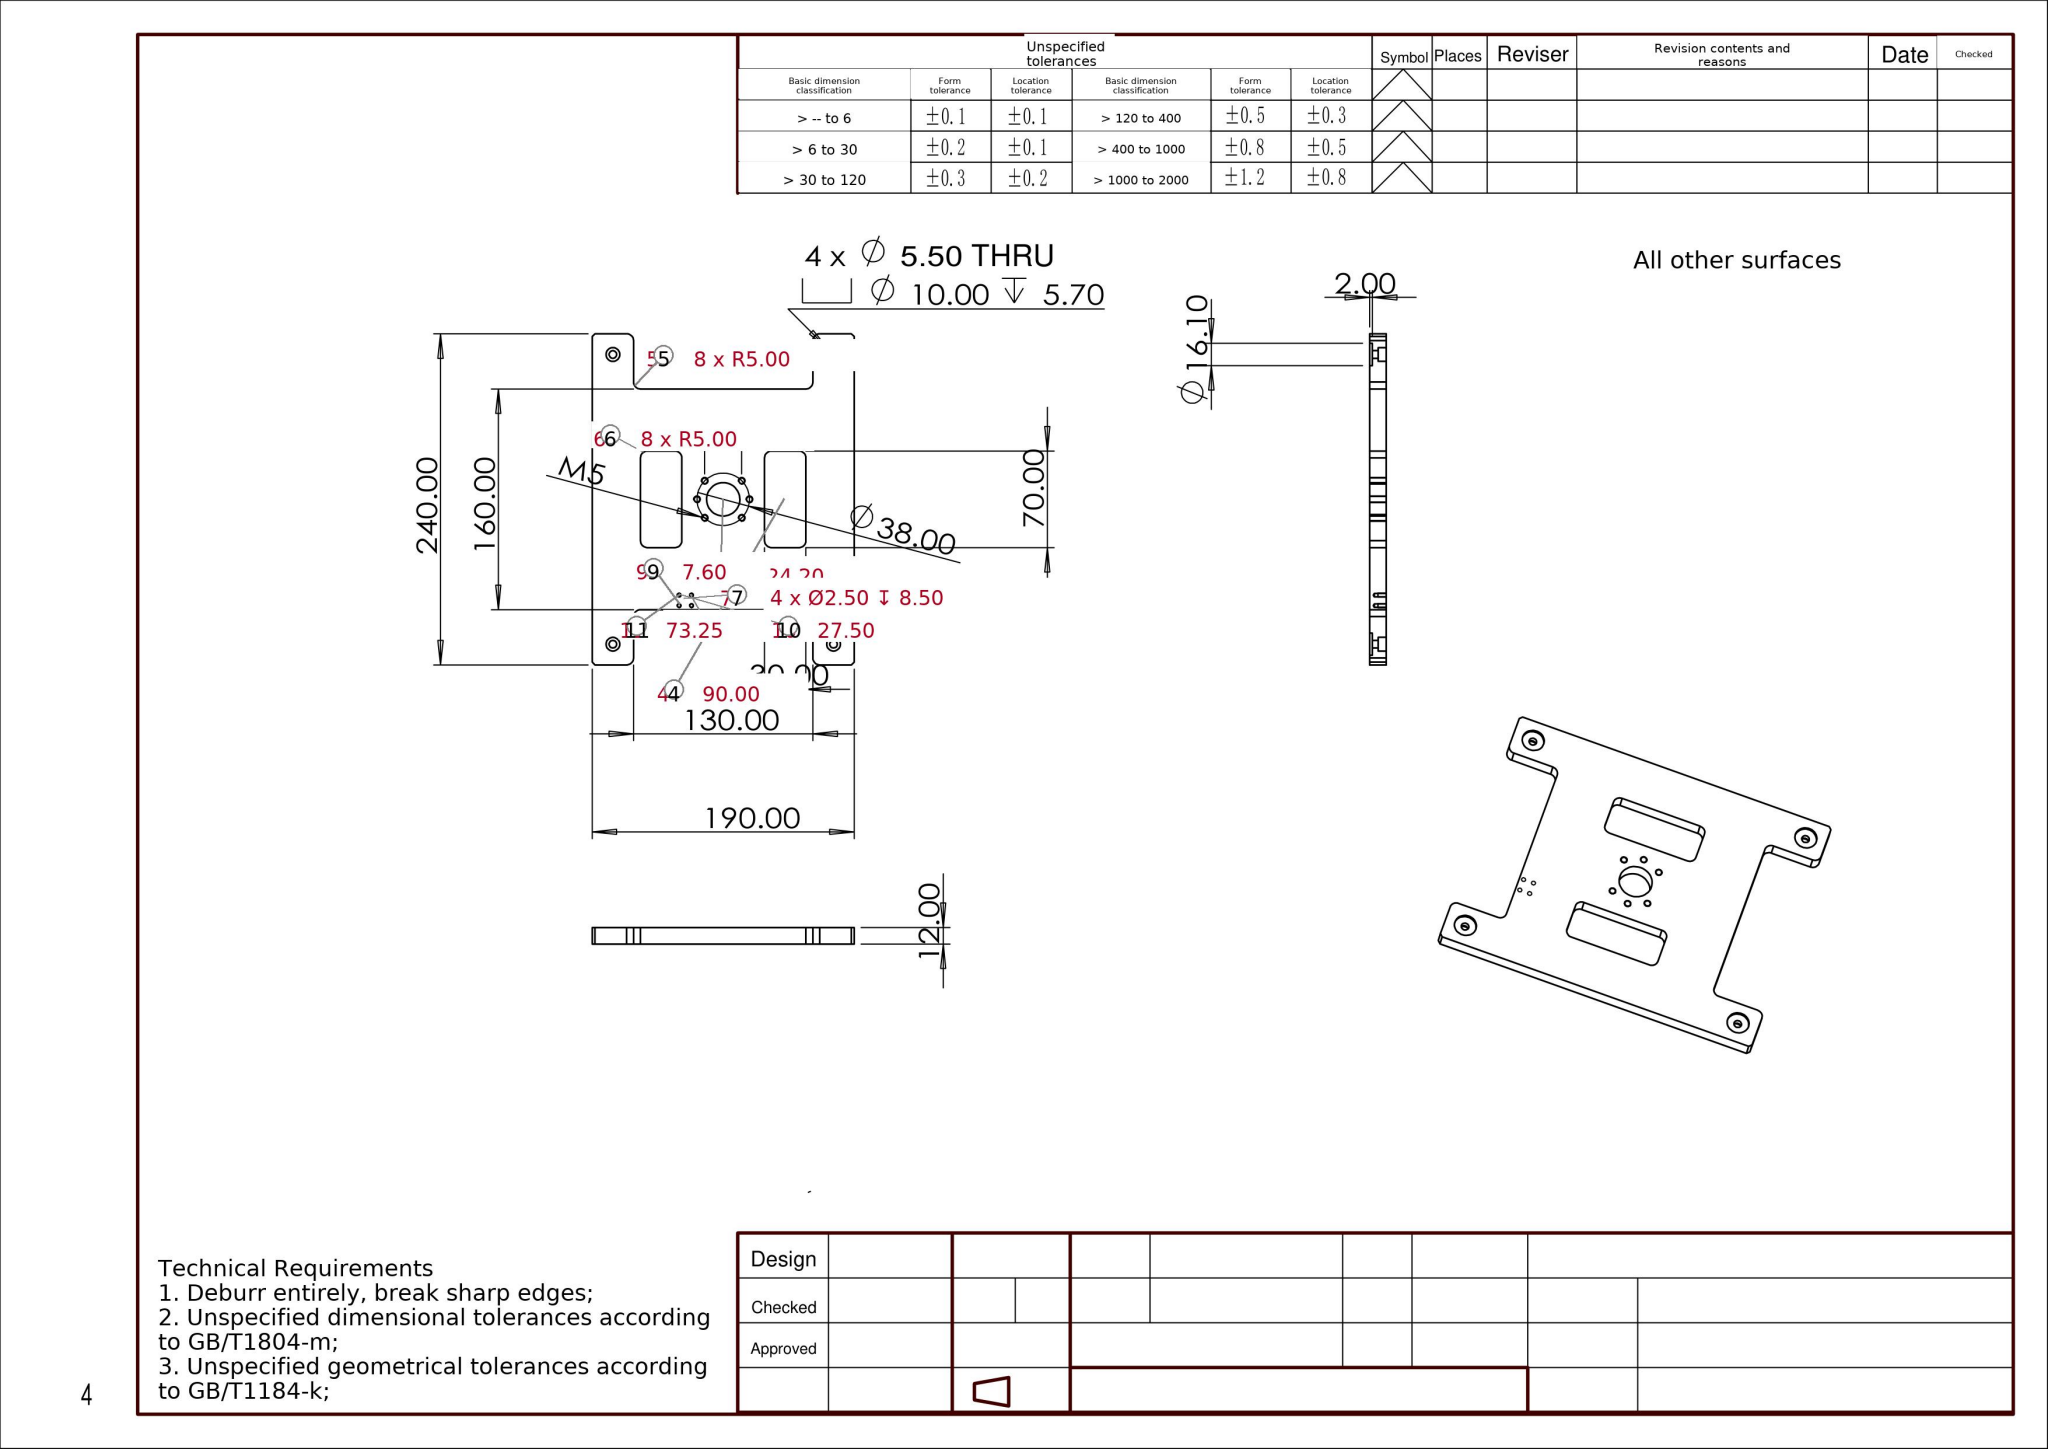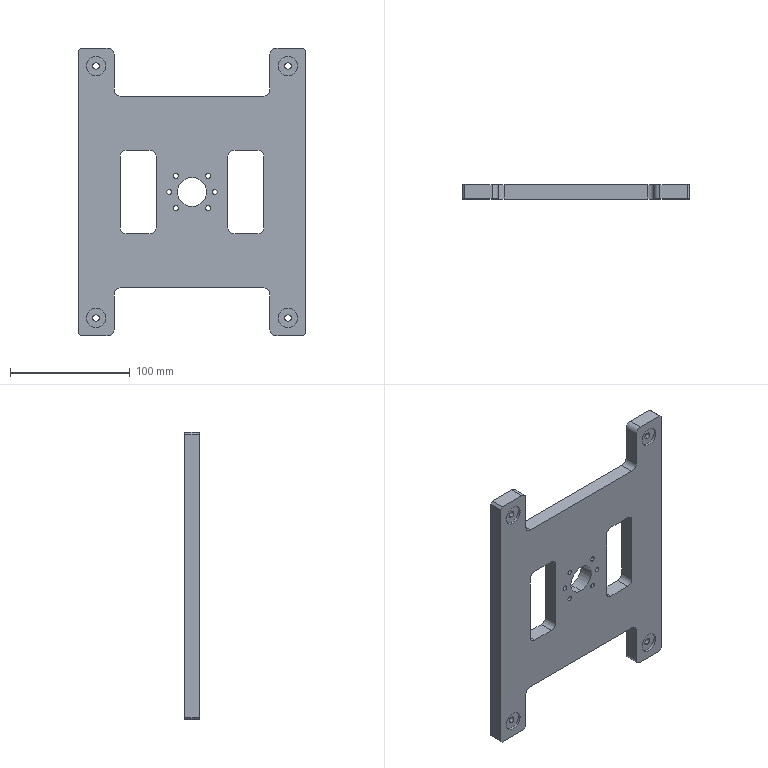Part | SolidWorks | mm | 1 solid | 104 faces | box 190 x 12 x 240 mm | volume 361902 mm3 | cylinder 62 | plane 34 | cone 8 | commonest cylinder face diameters 10 x24 4.2 x12 2.5 x8 16.1 x8 5.5 x8 24.2 x2
build123d program:
from build123d import *

# Parameters (mm, degrees)
SKETCH1_W                                         = 190
SKETCH1_H                                         = 240
BOSS_EXTRUDE1_DEPTH                               = 6
SKETCH2_W                                         = 30
SKETCH2_H                                         = 70
CUT_EXTRUDE1_DEPTH                                = 154.522
HOLE_SIZE_ACCORDING_TO_HEXAGON_SOCKET_D           = 5.5
HOLE_SIZE_ACCORDING_TO_HEXAGON_SOCKET_CBORE_D     = 10
HOLE_SIZE_ACCORDING_TO_HEXAGON_SOCKET_CBORE_DEPTH = 5.7
SKETCH5_R                                         = 12.1
CUT_EXTRUDE2_DEPTH                                = 154.522
FILLET1_R                                         = 5
CHAMFER1_SIZE                                     = 2
SKETCH12_R                                        = 8.05
CUT_EXTRUDE3_DEPTH                                = 2
SKETCH17_W                                        = 130
SKETCH17_H                                        = 80
CUT_EXTRUDE4_DEPTH                                = 154.522
M3_TAPPED_HOLE1_D                                 = 2.5
M3_TAPPED_HOLE1_DEPTH                             = 8.5
M3_TAPPED_HOLE1_TIP                               = 0.7511
FILLET2_R                                         = 5
M5_TAPPED_HOLE1_D                                 = 4.2


with BuildPart() as part:
    # Sketch1 → Boss-Extrude1 (new, symmetric)
    with BuildSketch(Plane(origin=(0, 0, 0), x_dir=(1, 0, 0), z_dir=(0, 1, 0))):
        Rectangle(SKETCH1_W, SKETCH1_H)
    extrude(amount=BOSS_EXTRUDE1_DEPTH, both=True)

    # Sketch2 → Cut-Extrude1 (cut, through all)
    with BuildSketch(Plane(origin=(0, 6, 0), x_dir=(1, 0, 0), z_dir=(0, 1, 0))):
        with Locations((-45, 0)):
            Rectangle(SKETCH2_W, SKETCH2_H)
        with Locations((45, 0)):
            Rectangle(SKETCH2_W, SKETCH2_H)
    extrude(amount=-CUT_EXTRUDE1_DEPTH, mode=Mode.SUBTRACT)

    # Hole Size _According to_ Hexagon Socket (through all)
    with Locations(Plane(origin=(0, 6, 0), x_dir=(-1, 0, 0), z_dir=(0, 1, 0))):
        with Locations((80, -105), (80, 105), (-80, -105), (-80, 105)):
            CounterBoreHole(HOLE_SIZE_ACCORDING_TO_HEXAGON_SOCKET_D / 2, HOLE_SIZE_ACCORDING_TO_HEXAGON_SOCKET_CBORE_D / 2, HOLE_SIZE_ACCORDING_TO_HEXAGON_SOCKET_CBORE_DEPTH)

    # Sketch5 → Cut-Extrude2 (cut, through all)
    with BuildSketch(Plane.XZ.offset(6)):
        with Locations(Location((0, 0, 0), (0, 0, 270))):
            Circle(SKETCH5_R)
    extrude(amount=-CUT_EXTRUDE2_DEPTH, mode=Mode.SUBTRACT)

    # Fillet1
    fillet1_edges = [part.edges().sort_by_distance(p)[0] for p in [
        (-60, 0, 35),
        (-60, 0, -35),
        (-30, 0, -35),
        (-30, 0, 35),
        (30, 0, 35),
        (30, 0, -35),
        (60, 0, -35),
        (60, 0, 35),
    ]]
    fillet(fillet1_edges, radius=FILLET1_R)

    # Chamfer1
    chamfer1_edges = [part.edges().sort_by_distance(p)[0] for p in [
        (-95, 0, -120),
        (95, 0, -120),
        (95, 0, 120),
        (-95, 0, 120),
    ]]
    chamfer(chamfer1_edges, length=CHAMFER1_SIZE)

    # Sketch12 → Cut-Extrude3 (cut)
    with BuildSketch(Plane.XZ.offset(6)):
        with Locations(Location((-80, 105, 0), (0, 0, 270))):
            Circle(SKETCH12_R)
        with Locations(Location((-80, -105, 0), (0, 0, 90))):
            Circle(SKETCH12_R)
        with Locations(Location((80, -105, 0), (0, 0, 270))):
            Circle(SKETCH12_R)
        with Locations(Location((80, 105, 0), (0, 0, 90))):
            Circle(SKETCH12_R)
    extrude(amount=-CUT_EXTRUDE3_DEPTH, mode=Mode.SUBTRACT)

    # Sketch17 → Cut-Extrude4 (cut, through all)
    with BuildSketch(Plane(origin=(0, 6, 0), x_dir=(1, 0, 0), z_dir=(0, 1, 0))):
        with Locations((0, -120)):
            Rectangle(SKETCH17_W, SKETCH17_H)
    cut_extrude4 = extrude(amount=-CUT_EXTRUDE4_DEPTH, mode=Mode.SUBTRACT)

    # M3 Tapped Hole1
    with Locations(Plane(origin=(0, 6, 0), x_dir=(-1, 0, 0), z_dir=(0, 1, 0))):
        with Locations((23, 69.45), (23, 77.05), (32, 77.05), (32, 69.45)):
            Hole(M3_TAPPED_HOLE1_D / 2, depth=M3_TAPPED_HOLE1_DEPTH)
            with Locations((0, 0, -(M3_TAPPED_HOLE1_DEPTH + M3_TAPPED_HOLE1_TIP / 2))):  # 118° drill point
                Cone(0, M3_TAPPED_HOLE1_D / 2, M3_TAPPED_HOLE1_TIP, mode=Mode.SUBTRACT)

    # Mirror1: Cut-Extrude4 across plane
    add(cut_extrude4.mirror(Plane.XY), mode=Mode.SUBTRACT)

    # Fillet2
    fillet2_edges = [part.edges().sort_by_distance(p)[0] for p in [
        (65, 0, 120),
        (65, 0, 80),
        (-65, 0, 120),
        (-65, 0, 80),
        (-65, 0, -80),
        (65, 0, -120),
        (65, 0, -80),
        (-65, 0, -120),
    ]]
    fillet(fillet2_edges, radius=FILLET2_R)

    # M5 Tapped Hole1 (through all)
    with Locations(Plane(origin=(0, -6, 0), x_dir=(-1, 0, 0), z_dir=(0, -1, 0))):
        with Locations((-13.435, 13.435), (-19, 0), (-13.435, -13.435), (13.435, -13.435), (19, 0), (13.435, 13.435)):
            Hole(M5_TAPPED_HOLE1_D / 2)


solid = part.part